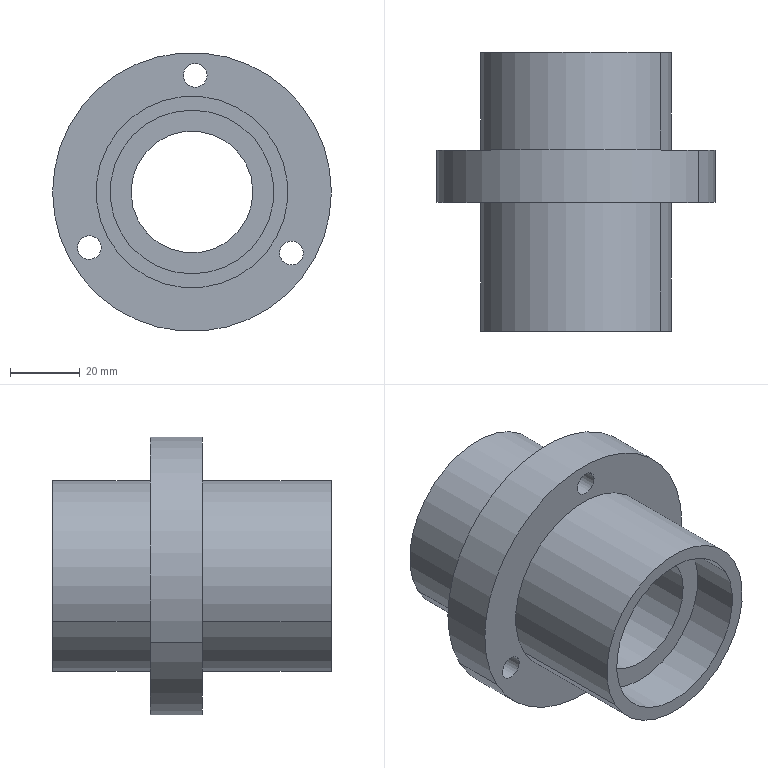Component | SolidWorks | BearingHousing1-1 | 1 solid | 24 faces | box 80 x 80 x 80 mm | volume 129585 mm3 | cylinder 18 | plane 6 | commonest cylinder face diameters 6.8 x6 47 x4 55 x4 35 x2 80 x2
STEP:
#1=CARTESIAN_POINT('',(-9.498,17.558,-6.667));
#2=VERTEX_POINT('',#1);
#3=CARTESIAN_POINT('',(-9.733,17.558,-6.794));
#4=VERTEX_POINT('',#3);
#5=CARTESIAN_POINT('',(-9.616,17.558,-6.73));
#6=DIRECTION('',(0.,-1.,0.));
#7=DIRECTION('',(-0.8793,0.,-0.4762));
#8=AXIS2_PLACEMENT_3D('',#5,#6,#7);
#9=CIRCLE('',#8,0.1339);
#10=EDGE_CURVE('',#2,#4,#9,.T.);
#11=ORIENTED_EDGE('',*,*,#10,.T.);
#12=CARTESIAN_POINT('',(-9.733,18.149,-6.794));
#13=VERTEX_POINT('',#12);
#14=CARTESIAN_POINT('',(-9.733,18.149,-6.794));
#15=DIRECTION('',(0.,1.,0.));
#16=VECTOR('',#15,39.37);
#17=LINE('',#14,#16);
#18=EDGE_CURVE('',#4,#13,#17,.T.);
#19=ORIENTED_EDGE('',*,*,#18,.T.);
#20=CARTESIAN_POINT('',(-9.498,18.149,-6.667));
#21=VERTEX_POINT('',#20);
#22=CARTESIAN_POINT('',(-9.616,18.149,-6.73));
#23=DIRECTION('',(0.,1.,0.));
#24=DIRECTION('',(0.8793,0.,0.4762));
#25=AXIS2_PLACEMENT_3D('',#22,#23,#24);
#26=CIRCLE('',#25,0.1339);
#27=EDGE_CURVE('',#13,#21,#26,.T.);
#28=ORIENTED_EDGE('',*,*,#27,.T.);
#29=CARTESIAN_POINT('',(-9.498,18.149,-6.667));
#30=DIRECTION('',(0.,1.,0.));
#31=VECTOR('',#30,39.37);
#32=LINE('',#29,#31);
#33=EDGE_CURVE('',#2,#21,#32,.T.);
#34=ORIENTED_EDGE('',*,*,#33,.F.);
#35=EDGE_LOOP('',(#11,#19,#28,#34));
#36=FACE_OUTER_BOUND('',#35,.T.);
#37=CARTESIAN_POINT('',(-9.616,18.149,-6.73));
#38=DIRECTION('',(0.,1.,0.));
#39=DIRECTION('',(0.8793,0.,0.4762));
#40=AXIS2_PLACEMENT_3D('',#37,#38,#39);
#41=CYLINDRICAL_SURFACE('',#40,0.1339);
#42=ADVANCED_FACE('',(#36),#41,.F.);
#43=CARTESIAN_POINT('',(-8.302,17.558,-4.72));
#44=VERTEX_POINT('',#43);
#45=CARTESIAN_POINT('',(-8.538,17.558,-4.848));
#46=VERTEX_POINT('',#45);
#47=CARTESIAN_POINT('',(-8.42,17.558,-4.784));
#48=DIRECTION('',(0.,-1.,0.));
#49=DIRECTION('',(-0.8793,0.,-0.4762));
#50=AXIS2_PLACEMENT_3D('',#47,#48,#49);
#51=CIRCLE('',#50,0.1339);
#52=EDGE_CURVE('',#44,#46,#51,.T.);
#53=ORIENTED_EDGE('',*,*,#52,.T.);
#54=CARTESIAN_POINT('',(-8.538,18.149,-4.848));
#55=VERTEX_POINT('',#54);
#56=CARTESIAN_POINT('',(-8.538,18.149,-4.848));
#57=DIRECTION('',(0.,1.,0.));
#58=VECTOR('',#57,39.37);
#59=LINE('',#56,#58);
#60=EDGE_CURVE('',#46,#55,#59,.T.);
#61=ORIENTED_EDGE('',*,*,#60,.T.);
#62=CARTESIAN_POINT('',(-8.302,18.149,-4.72));
#63=VERTEX_POINT('',#62);
#64=CARTESIAN_POINT('',(-8.42,18.149,-4.784));
#65=DIRECTION('',(0.,1.,0.));
#66=DIRECTION('',(0.8793,0.,0.4762));
#67=AXIS2_PLACEMENT_3D('',#64,#65,#66);
#68=CIRCLE('',#67,0.1339);
#69=EDGE_CURVE('',#55,#63,#68,.T.);
#70=ORIENTED_EDGE('',*,*,#69,.T.);
#71=CARTESIAN_POINT('',(-8.302,18.149,-4.72));
#72=DIRECTION('',(0.,1.,0.));
#73=VECTOR('',#72,39.37);
#74=LINE('',#71,#73);
#75=EDGE_CURVE('',#44,#63,#74,.T.);
#76=ORIENTED_EDGE('',*,*,#75,.F.);
#77=EDGE_LOOP('',(#53,#61,#70,#76));
#78=FACE_OUTER_BOUND('',#77,.T.);
#79=CARTESIAN_POINT('',(-8.42,18.149,-4.784));
#80=DIRECTION('',(0.,1.,0.));
#81=DIRECTION('',(0.8793,0.,0.4762));
#82=AXIS2_PLACEMENT_3D('',#79,#80,#81);
#83=CYLINDRICAL_SURFACE('',#82,0.1339);
#84=ADVANCED_FACE('',(#78),#83,.F.);
#85=CARTESIAN_POINT('',(-7.215,17.558,-6.729));
#86=VERTEX_POINT('',#85);
#87=CARTESIAN_POINT('',(-7.45,17.558,-6.856));
#88=VERTEX_POINT('',#87);
#89=CARTESIAN_POINT('',(-7.332,17.558,-6.793));
#90=DIRECTION('',(0.,-1.,0.));
#91=DIRECTION('',(-0.8793,0.,-0.4762));
#92=AXIS2_PLACEMENT_3D('',#89,#90,#91);
#93=CIRCLE('',#92,0.1339);
#94=EDGE_CURVE('',#86,#88,#93,.T.);
#95=ORIENTED_EDGE('',*,*,#94,.T.);
#96=CARTESIAN_POINT('',(-7.45,18.149,-6.856));
#97=VERTEX_POINT('',#96);
#98=CARTESIAN_POINT('',(-7.45,18.149,-6.856));
#99=DIRECTION('',(0.,1.,0.));
#100=VECTOR('',#99,39.37);
#101=LINE('',#98,#100);
#102=EDGE_CURVE('',#88,#97,#101,.T.);
#103=ORIENTED_EDGE('',*,*,#102,.T.);
#104=CARTESIAN_POINT('',(-7.215,18.149,-6.729));
#105=VERTEX_POINT('',#104);
#106=CARTESIAN_POINT('',(-7.332,18.149,-6.793));
#107=DIRECTION('',(0.,1.,0.));
#108=DIRECTION('',(0.8793,0.,0.4762));
#109=AXIS2_PLACEMENT_3D('',#106,#107,#108);
#110=CIRCLE('',#109,0.1339);
#111=EDGE_CURVE('',#97,#105,#110,.T.);
#112=ORIENTED_EDGE('',*,*,#111,.T.);
#113=CARTESIAN_POINT('',(-7.215,18.149,-6.729));
#114=DIRECTION('',(0.,1.,0.));
#115=VECTOR('',#114,39.37);
#116=LINE('',#113,#115);
#117=EDGE_CURVE('',#86,#105,#116,.T.);
#118=ORIENTED_EDGE('',*,*,#117,.F.);
#119=EDGE_LOOP('',(#95,#103,#112,#118));
#120=FACE_OUTER_BOUND('',#119,.T.);
#121=CARTESIAN_POINT('',(-7.332,18.149,-6.793));
#122=DIRECTION('',(0.,1.,0.));
#123=DIRECTION('',(0.8793,0.,0.4762));
#124=AXIS2_PLACEMENT_3D('',#121,#122,#123);
#125=CYLINDRICAL_SURFACE('',#124,0.1339);
#126=ADVANCED_FACE('',(#120),#125,.F.);
#127=CARTESIAN_POINT('',(-7.85,18.7,-5.774));
#128=VERTEX_POINT('',#127);
#129=CARTESIAN_POINT('',(-9.062,18.7,-6.43));
#130=VERTEX_POINT('',#129);
#131=CARTESIAN_POINT('',(-8.456,18.7,-6.102));
#132=DIRECTION('',(0.,-1.,0.));
#133=DIRECTION('',(-0.8793,0.,-0.4762));
#134=AXIS2_PLACEMENT_3D('',#131,#132,#133);
#135=CIRCLE('',#134,0.689);
#136=EDGE_CURVE('',#128,#130,#135,.T.);
#137=ORIENTED_EDGE('',*,*,#136,.F.);
#138=CARTESIAN_POINT('',(-7.85,16.653,-5.774));
#139=VERTEX_POINT('',#138);
#140=CARTESIAN_POINT('',(-7.85,17.335,-5.774));
#141=DIRECTION('',(0.,-1.,0.));
#142=VECTOR('',#141,39.37);
#143=LINE('',#140,#142);
#144=EDGE_CURVE('',#128,#139,#143,.T.);
#145=ORIENTED_EDGE('',*,*,#144,.T.);
#146=CARTESIAN_POINT('',(-9.062,16.653,-6.43));
#147=VERTEX_POINT('',#146);
#148=CARTESIAN_POINT('',(-8.456,16.653,-6.102));
#149=DIRECTION('',(0.,-1.,0.));
#150=DIRECTION('',(-0.8793,0.,-0.4762));
#151=AXIS2_PLACEMENT_3D('',#148,#149,#150);
#152=CIRCLE('',#151,0.689);
#153=EDGE_CURVE('',#139,#147,#152,.T.);
#154=ORIENTED_EDGE('',*,*,#153,.T.);
#155=CARTESIAN_POINT('',(-9.062,17.335,-6.43));
#156=DIRECTION('',(0.,-1.,0.));
#157=VECTOR('',#156,39.37);
#158=LINE('',#155,#157);
#159=EDGE_CURVE('',#130,#147,#158,.T.);
#160=ORIENTED_EDGE('',*,*,#159,.F.);
#161=EDGE_LOOP('',(#137,#145,#154,#160));
#162=FACE_OUTER_BOUND('',#161,.T.);
#163=CARTESIAN_POINT('',(-8.456,17.335,-6.102));
#164=DIRECTION('',(0.,-1.,0.));
#165=DIRECTION('',(-0.8793,0.,-0.4762));
#166=AXIS2_PLACEMENT_3D('',#163,#164,#165);
#167=CYLINDRICAL_SURFACE('',#166,0.689);
#168=ADVANCED_FACE('',(#162),#167,.F.);
#169=CARTESIAN_POINT('',(-7.643,19.251,-5.662));
#170=VERTEX_POINT('',#169);
#171=CARTESIAN_POINT('',(-9.27,19.251,-6.543));
#172=VERTEX_POINT('',#171);
#173=CARTESIAN_POINT('',(-8.456,19.251,-6.102));
#174=DIRECTION('',(0.,-1.,0.));
#175=DIRECTION('',(-0.8793,0.,-0.4762));
#176=AXIS2_PLACEMENT_3D('',#173,#174,#175);
#177=CIRCLE('',#176,0.9252);
#178=EDGE_CURVE('',#170,#172,#177,.T.);
#179=ORIENTED_EDGE('',*,*,#178,.F.);
#180=CARTESIAN_POINT('',(-7.643,18.7,-5.662));
#181=VERTEX_POINT('',#180);
#182=CARTESIAN_POINT('',(-7.643,17.335,-5.662));
#183=DIRECTION('',(0.,-1.,0.));
#184=VECTOR('',#183,39.37);
#185=LINE('',#182,#184);
#186=EDGE_CURVE('',#170,#181,#185,.T.);
#187=ORIENTED_EDGE('',*,*,#186,.T.);
#188=CARTESIAN_POINT('',(-9.27,18.7,-6.543));
#189=VERTEX_POINT('',#188);
#190=CARTESIAN_POINT('',(-8.456,18.7,-6.102));
#191=DIRECTION('',(0.,-1.,0.));
#192=DIRECTION('',(-0.8793,0.,-0.4762));
#193=AXIS2_PLACEMENT_3D('',#190,#191,#192);
#194=CIRCLE('',#193,0.9252);
#195=EDGE_CURVE('',#181,#189,#194,.T.);
#196=ORIENTED_EDGE('',*,*,#195,.T.);
#197=CARTESIAN_POINT('',(-9.27,17.335,-6.543));
#198=DIRECTION('',(0.,-1.,0.));
#199=VECTOR('',#198,39.37);
#200=LINE('',#197,#199);
#201=EDGE_CURVE('',#172,#189,#200,.T.);
#202=ORIENTED_EDGE('',*,*,#201,.F.);
#203=EDGE_LOOP('',(#179,#187,#196,#202));
#204=FACE_OUTER_BOUND('',#203,.T.);
#205=CARTESIAN_POINT('',(-8.456,17.335,-6.102));
#206=DIRECTION('',(0.,-1.,0.));
#207=DIRECTION('',(-0.8793,0.,-0.4762));
#208=AXIS2_PLACEMENT_3D('',#205,#206,#207);
#209=CYLINDRICAL_SURFACE('',#208,0.9252);
#210=ADVANCED_FACE('',(#204),#209,.F.);
#211=CARTESIAN_POINT('',(-9.408,19.251,-6.618));
#212=VERTEX_POINT('',#211);
#213=CARTESIAN_POINT('',(-7.504,19.251,-5.587));
#214=VERTEX_POINT('',#213);
#215=CARTESIAN_POINT('',(-8.456,19.251,-6.102));
#216=DIRECTION('',(0.,-1.,0.));
#217=DIRECTION('',(-0.8793,0.,-0.4762));
#218=AXIS2_PLACEMENT_3D('',#215,#216,#217);
#219=CIRCLE('',#218,1.083);
#220=EDGE_CURVE('',#212,#214,#219,.T.);
#221=ORIENTED_EDGE('',*,*,#220,.T.);
#222=CARTESIAN_POINT('',(-7.504,18.149,-5.587));
#223=VERTEX_POINT('',#222);
#224=CARTESIAN_POINT('',(-7.504,17.335,-5.587));
#225=DIRECTION('',(0.,-1.,0.));
#226=VECTOR('',#225,39.37);
#227=LINE('',#224,#226);
#228=EDGE_CURVE('',#214,#223,#227,.T.);
#229=ORIENTED_EDGE('',*,*,#228,.T.);
#230=CARTESIAN_POINT('',(-9.408,18.149,-6.618));
#231=VERTEX_POINT('',#230);
#232=CARTESIAN_POINT('',(-8.456,18.149,-6.102));
#233=DIRECTION('',(0.,-1.,0.));
#234=DIRECTION('',(-0.8793,0.,-0.4762));
#235=AXIS2_PLACEMENT_3D('',#232,#233,#234);
#236=CIRCLE('',#235,1.083);
#237=EDGE_CURVE('',#231,#223,#236,.T.);
#238=ORIENTED_EDGE('',*,*,#237,.F.);
#239=CARTESIAN_POINT('',(-9.408,17.335,-6.618));
#240=DIRECTION('',(0.,-1.,0.));
#241=VECTOR('',#240,39.37);
#242=LINE('',#239,#241);
#243=EDGE_CURVE('',#212,#231,#242,.T.);
#244=ORIENTED_EDGE('',*,*,#243,.F.);
#245=EDGE_LOOP('',(#221,#229,#238,#244));
#246=FACE_OUTER_BOUND('',#245,.T.);
#247=CARTESIAN_POINT('',(-8.456,17.335,-6.102));
#248=DIRECTION('',(0.,-1.,0.));
#249=DIRECTION('',(-0.8793,0.,-0.4762));
#250=AXIS2_PLACEMENT_3D('',#247,#248,#249);
#251=CYLINDRICAL_SURFACE('',#250,1.083);
#252=ADVANCED_FACE('',(#246),#251,.T.);
#253=CARTESIAN_POINT('',(-9.841,18.149,-6.852));
#254=VERTEX_POINT('',#253);
#255=CARTESIAN_POINT('',(-7.071,18.149,-5.352));
#256=VERTEX_POINT('',#255);
#257=CARTESIAN_POINT('',(-8.456,18.149,-6.102));
#258=DIRECTION('',(0.,-1.,0.));
#259=DIRECTION('',(-0.8793,0.,-0.4762));
#260=AXIS2_PLACEMENT_3D('',#257,#258,#259);
#261=CIRCLE('',#260,1.575);
#262=EDGE_CURVE('',#254,#256,#261,.T.);
#263=ORIENTED_EDGE('',*,*,#262,.T.);
#264=CARTESIAN_POINT('',(-7.071,17.558,-5.352));
#265=VERTEX_POINT('',#264);
#266=CARTESIAN_POINT('',(-7.071,17.335,-5.352));
#267=DIRECTION('',(0.,-1.,0.));
#268=VECTOR('',#267,39.37);
#269=LINE('',#266,#268);
#270=EDGE_CURVE('',#256,#265,#269,.T.);
#271=ORIENTED_EDGE('',*,*,#270,.T.);
#272=CARTESIAN_POINT('',(-9.841,17.558,-6.852));
#273=VERTEX_POINT('',#272);
#274=CARTESIAN_POINT('',(-8.456,17.558,-6.102));
#275=DIRECTION('',(0.,-1.,0.));
#276=DIRECTION('',(-0.8793,0.,-0.4762));
#277=AXIS2_PLACEMENT_3D('',#274,#275,#276);
#278=CIRCLE('',#277,1.575);
#279=EDGE_CURVE('',#273,#265,#278,.T.);
#280=ORIENTED_EDGE('',*,*,#279,.F.);
#281=CARTESIAN_POINT('',(-9.841,17.335,-6.852));
#282=DIRECTION('',(0.,-1.,0.));
#283=VECTOR('',#282,39.37);
#284=LINE('',#281,#283);
#285=EDGE_CURVE('',#254,#273,#284,.T.);
#286=ORIENTED_EDGE('',*,*,#285,.F.);
#287=EDGE_LOOP('',(#263,#271,#280,#286));
#288=FACE_OUTER_BOUND('',#287,.T.);
#289=CARTESIAN_POINT('',(-8.456,17.335,-6.102));
#290=DIRECTION('',(0.,-1.,0.));
#291=DIRECTION('',(-0.8793,0.,-0.4762));
#292=AXIS2_PLACEMENT_3D('',#289,#290,#291);
#293=CYLINDRICAL_SURFACE('',#292,1.575);
#294=ADVANCED_FACE('',(#288),#293,.T.);
#295=CARTESIAN_POINT('',(-9.408,17.558,-6.618));
#296=VERTEX_POINT('',#295);
#297=CARTESIAN_POINT('',(-7.504,17.558,-5.587));
#298=VERTEX_POINT('',#297);
#299=CARTESIAN_POINT('',(-8.456,17.558,-6.102));
#300=DIRECTION('',(0.,-1.,0.));
#301=DIRECTION('',(-0.8793,0.,-0.4762));
#302=AXIS2_PLACEMENT_3D('',#299,#300,#301);
#303=CIRCLE('',#302,1.083);
#304=EDGE_CURVE('',#296,#298,#303,.T.);
#305=ORIENTED_EDGE('',*,*,#304,.T.);
#306=CARTESIAN_POINT('',(-7.504,16.102,-5.587));
#307=VERTEX_POINT('',#306);
#308=CARTESIAN_POINT('',(-7.504,17.335,-5.587));
#309=DIRECTION('',(0.,-1.,0.));
#310=VECTOR('',#309,39.37);
#311=LINE('',#308,#310);
#312=EDGE_CURVE('',#298,#307,#311,.T.);
#313=ORIENTED_EDGE('',*,*,#312,.T.);
#314=CARTESIAN_POINT('',(-9.408,16.102,-6.618));
#315=VERTEX_POINT('',#314);
#316=CARTESIAN_POINT('',(-8.456,16.102,-6.102));
#317=DIRECTION('',(0.,-1.,0.));
#318=DIRECTION('',(-0.8793,0.,-0.4762));
#319=AXIS2_PLACEMENT_3D('',#316,#317,#318);
#320=CIRCLE('',#319,1.083);
#321=EDGE_CURVE('',#315,#307,#320,.T.);
#322=ORIENTED_EDGE('',*,*,#321,.F.);
#323=CARTESIAN_POINT('',(-9.408,17.335,-6.618));
#324=DIRECTION('',(0.,-1.,0.));
#325=VECTOR('',#324,39.37);
#326=LINE('',#323,#325);
#327=EDGE_CURVE('',#296,#315,#326,.T.);
#328=ORIENTED_EDGE('',*,*,#327,.F.);
#329=EDGE_LOOP('',(#305,#313,#322,#328));
#330=FACE_OUTER_BOUND('',#329,.T.);
#331=CARTESIAN_POINT('',(-8.456,17.335,-6.102));
#332=DIRECTION('',(0.,-1.,0.));
#333=DIRECTION('',(-0.8793,0.,-0.4762));
#334=AXIS2_PLACEMENT_3D('',#331,#332,#333);
#335=CYLINDRICAL_SURFACE('',#334,1.083);
#336=ADVANCED_FACE('',(#330),#335,.T.);
#337=CARTESIAN_POINT('',(-7.643,16.653,-5.662));
#338=VERTEX_POINT('',#337);
#339=CARTESIAN_POINT('',(-9.27,16.653,-6.543));
#340=VERTEX_POINT('',#339);
#341=CARTESIAN_POINT('',(-8.456,16.653,-6.102));
#342=DIRECTION('',(0.,-1.,0.));
#343=DIRECTION('',(-0.8793,0.,-0.4762));
#344=AXIS2_PLACEMENT_3D('',#341,#342,#343);
#345=CIRCLE('',#344,0.9252);
#346=EDGE_CURVE('',#338,#340,#345,.T.);
#347=ORIENTED_EDGE('',*,*,#346,.F.);
#348=CARTESIAN_POINT('',(-7.643,16.102,-5.662));
#349=VERTEX_POINT('',#348);
#350=CARTESIAN_POINT('',(-7.643,17.335,-5.662));
#351=DIRECTION('',(0.,-1.,0.));
#352=VECTOR('',#351,39.37);
#353=LINE('',#350,#352);
#354=EDGE_CURVE('',#338,#349,#353,.T.);
#355=ORIENTED_EDGE('',*,*,#354,.T.);
#356=CARTESIAN_POINT('',(-9.27,16.102,-6.543));
#357=VERTEX_POINT('',#356);
#358=CARTESIAN_POINT('',(-8.456,16.102,-6.102));
#359=DIRECTION('',(0.,-1.,0.));
#360=DIRECTION('',(-0.8793,0.,-0.4762));
#361=AXIS2_PLACEMENT_3D('',#358,#359,#360);
#362=CIRCLE('',#361,0.9252);
#363=EDGE_CURVE('',#349,#357,#362,.T.);
#364=ORIENTED_EDGE('',*,*,#363,.T.);
#365=CARTESIAN_POINT('',(-9.27,17.335,-6.543));
#366=DIRECTION('',(0.,-1.,0.));
#367=VECTOR('',#366,39.37);
#368=LINE('',#365,#367);
#369=EDGE_CURVE('',#340,#357,#368,.T.);
#370=ORIENTED_EDGE('',*,*,#369,.F.);
#371=EDGE_LOOP('',(#347,#355,#364,#370));
#372=FACE_OUTER_BOUND('',#371,.T.);
#373=CARTESIAN_POINT('',(-8.456,17.335,-6.102));
#374=DIRECTION('',(0.,-1.,0.));
#375=DIRECTION('',(-0.8793,0.,-0.4762));
#376=AXIS2_PLACEMENT_3D('',#373,#374,#375);
#377=CYLINDRICAL_SURFACE('',#376,0.9252);
#378=ADVANCED_FACE('',(#372),#377,.F.);
#379=ORIENTED_EDGE('',*,*,#354,.F.);
#380=CARTESIAN_POINT('',(-8.456,16.653,-6.102));
#381=DIRECTION('',(0.,-1.,0.));
#382=DIRECTION('',(-0.8793,0.,-0.4762));
#383=AXIS2_PLACEMENT_3D('',#380,#381,#382);
#384=CIRCLE('',#383,0.9252);
#385=EDGE_CURVE('',#340,#338,#384,.T.);
#386=ORIENTED_EDGE('',*,*,#385,.F.);
#387=ORIENTED_EDGE('',*,*,#369,.T.);
#388=CARTESIAN_POINT('',(-8.456,16.102,-6.102));
#389=DIRECTION('',(0.,-1.,0.));
#390=DIRECTION('',(-0.8793,0.,-0.4762));
#391=AXIS2_PLACEMENT_3D('',#388,#389,#390);
#392=CIRCLE('',#391,0.9252);
#393=EDGE_CURVE('',#357,#349,#392,.T.);
#394=ORIENTED_EDGE('',*,*,#393,.T.);
#395=EDGE_LOOP('',(#379,#386,#387,#394));
#396=FACE_OUTER_BOUND('',#395,.T.);
#397=CARTESIAN_POINT('',(-8.456,17.335,-6.102));
#398=DIRECTION('',(0.,-1.,0.));
#399=DIRECTION('',(-0.8793,0.,-0.4762));
#400=AXIS2_PLACEMENT_3D('',#397,#398,#399);
#401=CYLINDRICAL_SURFACE('',#400,0.9252);
#402=ADVANCED_FACE('',(#396),#401,.F.);
#403=ORIENTED_EDGE('',*,*,#321,.T.);
#404=CARTESIAN_POINT('',(-8.456,16.102,-6.102));
#405=DIRECTION('',(0.,-1.,0.));
#406=DIRECTION('',(-0.8793,0.,-0.4762));
#407=AXIS2_PLACEMENT_3D('',#404,#405,#406);
#408=CIRCLE('',#407,1.083);
#409=EDGE_CURVE('',#307,#315,#408,.T.);
#410=ORIENTED_EDGE('',*,*,#409,.T.);
#411=EDGE_LOOP('',(#403,#410));
#412=FACE_OUTER_BOUND('',#411,.T.);
#413=ORIENTED_EDGE('',*,*,#393,.F.);
#414=ORIENTED_EDGE('',*,*,#363,.F.);
#415=EDGE_LOOP('',(#413,#414));
#416=FACE_BOUND('',#415,.T.);
#417=CARTESIAN_POINT('',(-9.408,16.102,-6.618));
#418=DIRECTION('',(0.,-1.,0.));
#419=DIRECTION('',(-0.8793,-0.,-0.4762));
#420=AXIS2_PLACEMENT_3D('',#417,#418,#419);
#421=PLANE('',#420);
#422=ADVANCED_FACE('',(#412,#416),#421,.T.);
#423=ORIENTED_EDGE('',*,*,#312,.F.);
#424=CARTESIAN_POINT('',(-8.456,17.558,-6.102));
#425=DIRECTION('',(0.,-1.,0.));
#426=DIRECTION('',(-0.8793,0.,-0.4762));
#427=AXIS2_PLACEMENT_3D('',#424,#425,#426);
#428=CIRCLE('',#427,1.083);
#429=EDGE_CURVE('',#298,#296,#428,.T.);
#430=ORIENTED_EDGE('',*,*,#429,.T.);
#431=ORIENTED_EDGE('',*,*,#327,.T.);
#432=ORIENTED_EDGE('',*,*,#409,.F.);
#433=EDGE_LOOP('',(#423,#430,#431,#432));
#434=FACE_OUTER_BOUND('',#433,.T.);
#435=CARTESIAN_POINT('',(-8.456,17.335,-6.102));
#436=DIRECTION('',(0.,-1.,0.));
#437=DIRECTION('',(-0.8793,0.,-0.4762));
#438=AXIS2_PLACEMENT_3D('',#435,#436,#437);
#439=CYLINDRICAL_SURFACE('',#438,1.083);
#440=ADVANCED_FACE('',(#434),#439,.T.);
#441=ORIENTED_EDGE('',*,*,#10,.F.);
#442=CARTESIAN_POINT('',(-9.616,17.558,-6.73));
#443=DIRECTION('',(0.,-1.,0.));
#444=DIRECTION('',(-0.8793,0.,-0.4762));
#445=AXIS2_PLACEMENT_3D('',#442,#443,#444);
#446=CIRCLE('',#445,0.1339);
#447=EDGE_CURVE('',#4,#2,#446,.T.);
#448=ORIENTED_EDGE('',*,*,#447,.F.);
#449=EDGE_LOOP('',(#441,#448));
#450=FACE_BOUND('',#449,.T.);
#451=ORIENTED_EDGE('',*,*,#52,.F.);
#452=CARTESIAN_POINT('',(-8.42,17.558,-4.784));
#453=DIRECTION('',(0.,-1.,0.));
#454=DIRECTION('',(-0.8793,0.,-0.4762));
#455=AXIS2_PLACEMENT_3D('',#452,#453,#454);
#456=CIRCLE('',#455,0.1339);
#457=EDGE_CURVE('',#46,#44,#456,.T.);
#458=ORIENTED_EDGE('',*,*,#457,.F.);
#459=EDGE_LOOP('',(#451,#458));
#460=FACE_BOUND('',#459,.T.);
#461=ORIENTED_EDGE('',*,*,#94,.F.);
#462=CARTESIAN_POINT('',(-7.332,17.558,-6.793));
#463=DIRECTION('',(0.,-1.,0.));
#464=DIRECTION('',(-0.8793,0.,-0.4762));
#465=AXIS2_PLACEMENT_3D('',#462,#463,#464);
#466=CIRCLE('',#465,0.1339);
#467=EDGE_CURVE('',#88,#86,#466,.T.);
#468=ORIENTED_EDGE('',*,*,#467,.F.);
#469=EDGE_LOOP('',(#461,#468));
#470=FACE_BOUND('',#469,.T.);
#471=ORIENTED_EDGE('',*,*,#279,.T.);
#472=CARTESIAN_POINT('',(-8.456,17.558,-6.102));
#473=DIRECTION('',(0.,-1.,0.));
#474=DIRECTION('',(-0.8793,0.,-0.4762));
#475=AXIS2_PLACEMENT_3D('',#472,#473,#474);
#476=CIRCLE('',#475,1.575);
#477=EDGE_CURVE('',#265,#273,#476,.T.);
#478=ORIENTED_EDGE('',*,*,#477,.T.);
#479=EDGE_LOOP('',(#471,#478));
#480=FACE_OUTER_BOUND('',#479,.T.);
#481=ORIENTED_EDGE('',*,*,#304,.F.);
#482=ORIENTED_EDGE('',*,*,#429,.F.);
#483=EDGE_LOOP('',(#481,#482));
#484=FACE_BOUND('',#483,.T.);
#485=CARTESIAN_POINT('',(-9.841,17.558,-6.852));
#486=DIRECTION('',(0.,-1.,0.));
#487=DIRECTION('',(-0.8793,-0.,-0.4762));
#488=AXIS2_PLACEMENT_3D('',#485,#486,#487);
#489=PLANE('',#488);
#490=ADVANCED_FACE('',(#450,#460,#470,#480,#484),#489,.T.);
#491=ORIENTED_EDGE('',*,*,#270,.F.);
#492=CARTESIAN_POINT('',(-8.456,18.149,-6.102));
#493=DIRECTION('',(0.,-1.,0.));
#494=DIRECTION('',(-0.8793,0.,-0.4762));
#495=AXIS2_PLACEMENT_3D('',#492,#493,#494);
#496=CIRCLE('',#495,1.575);
#497=EDGE_CURVE('',#256,#254,#496,.T.);
#498=ORIENTED_EDGE('',*,*,#497,.T.);
#499=ORIENTED_EDGE('',*,*,#285,.T.);
#500=ORIENTED_EDGE('',*,*,#477,.F.);
#501=EDGE_LOOP('',(#491,#498,#499,#500));
#502=FACE_OUTER_BOUND('',#501,.T.);
#503=CARTESIAN_POINT('',(-8.456,17.335,-6.102));
#504=DIRECTION('',(0.,-1.,0.));
#505=DIRECTION('',(-0.8793,0.,-0.4762));
#506=AXIS2_PLACEMENT_3D('',#503,#504,#505);
#507=CYLINDRICAL_SURFACE('',#506,1.575);
#508=ADVANCED_FACE('',(#502),#507,.T.);
#509=CARTESIAN_POINT('',(-9.616,18.149,-6.73));
#510=DIRECTION('',(0.,1.,0.));
#511=DIRECTION('',(0.8793,0.,0.4762));
#512=AXIS2_PLACEMENT_3D('',#509,#510,#511);
#513=CIRCLE('',#512,0.1339);
#514=EDGE_CURVE('',#21,#13,#513,.T.);
#515=ORIENTED_EDGE('',*,*,#514,.F.);
#516=ORIENTED_EDGE('',*,*,#27,.F.);
#517=EDGE_LOOP('',(#515,#516));
#518=FACE_BOUND('',#517,.T.);
#519=CARTESIAN_POINT('',(-8.42,18.149,-4.784));
#520=DIRECTION('',(0.,1.,0.));
#521=DIRECTION('',(0.8793,0.,0.4762));
#522=AXIS2_PLACEMENT_3D('',#519,#520,#521);
#523=CIRCLE('',#522,0.1339);
#524=EDGE_CURVE('',#63,#55,#523,.T.);
#525=ORIENTED_EDGE('',*,*,#524,.F.);
#526=ORIENTED_EDGE('',*,*,#69,.F.);
#527=EDGE_LOOP('',(#525,#526));
#528=FACE_BOUND('',#527,.T.);
#529=CARTESIAN_POINT('',(-7.332,18.149,-6.793));
#530=DIRECTION('',(0.,1.,0.));
#531=DIRECTION('',(0.8793,0.,0.4762));
#532=AXIS2_PLACEMENT_3D('',#529,#530,#531);
#533=CIRCLE('',#532,0.1339);
#534=EDGE_CURVE('',#105,#97,#533,.T.);
#535=ORIENTED_EDGE('',*,*,#534,.F.);
#536=ORIENTED_EDGE('',*,*,#111,.F.);
#537=EDGE_LOOP('',(#535,#536));
#538=FACE_BOUND('',#537,.T.);
#539=ORIENTED_EDGE('',*,*,#237,.T.);
#540=CARTESIAN_POINT('',(-8.456,18.149,-6.102));
#541=DIRECTION('',(0.,-1.,0.));
#542=DIRECTION('',(-0.8793,0.,-0.4762));
#543=AXIS2_PLACEMENT_3D('',#540,#541,#542);
#544=CIRCLE('',#543,1.083);
#545=EDGE_CURVE('',#223,#231,#544,.T.);
#546=ORIENTED_EDGE('',*,*,#545,.T.);
#547=EDGE_LOOP('',(#539,#546));
#548=FACE_BOUND('',#547,.T.);
#549=ORIENTED_EDGE('',*,*,#262,.F.);
#550=ORIENTED_EDGE('',*,*,#497,.F.);
#551=EDGE_LOOP('',(#549,#550));
#552=FACE_OUTER_BOUND('',#551,.T.);
#553=CARTESIAN_POINT('',(-9.408,18.149,-6.618));
#554=DIRECTION('',(-0.,1.,-0.));
#555=DIRECTION('',(0.8793,0.,0.4762));
#556=AXIS2_PLACEMENT_3D('',#553,#554,#555);
#557=PLANE('',#556);
#558=ADVANCED_FACE('',(#518,#528,#538,#548,#552),#557,.T.);
#559=ORIENTED_EDGE('',*,*,#228,.F.);
#560=CARTESIAN_POINT('',(-8.456,19.251,-6.102));
#561=DIRECTION('',(0.,-1.,0.));
#562=DIRECTION('',(-0.8793,0.,-0.4762));
#563=AXIS2_PLACEMENT_3D('',#560,#561,#562);
#564=CIRCLE('',#563,1.083);
#565=EDGE_CURVE('',#214,#212,#564,.T.);
#566=ORIENTED_EDGE('',*,*,#565,.T.);
#567=ORIENTED_EDGE('',*,*,#243,.T.);
#568=ORIENTED_EDGE('',*,*,#545,.F.);
#569=EDGE_LOOP('',(#559,#566,#567,#568));
#570=FACE_OUTER_BOUND('',#569,.T.);
#571=CARTESIAN_POINT('',(-8.456,17.335,-6.102));
#572=DIRECTION('',(0.,-1.,0.));
#573=DIRECTION('',(-0.8793,0.,-0.4762));
#574=AXIS2_PLACEMENT_3D('',#571,#572,#573);
#575=CYLINDRICAL_SURFACE('',#574,1.083);
#576=ADVANCED_FACE('',(#570),#575,.T.);
#577=CARTESIAN_POINT('',(-8.456,19.251,-6.102));
#578=DIRECTION('',(0.,-1.,0.));
#579=DIRECTION('',(-0.8793,0.,-0.4762));
#580=AXIS2_PLACEMENT_3D('',#577,#578,#579);
#581=CIRCLE('',#580,0.9252);
#582=EDGE_CURVE('',#172,#170,#581,.T.);
#583=ORIENTED_EDGE('',*,*,#582,.T.);
#584=ORIENTED_EDGE('',*,*,#178,.T.);
#585=EDGE_LOOP('',(#583,#584));
#586=FACE_BOUND('',#585,.T.);
#587=ORIENTED_EDGE('',*,*,#220,.F.);
#588=ORIENTED_EDGE('',*,*,#565,.F.);
#589=EDGE_LOOP('',(#587,#588));
#590=FACE_OUTER_BOUND('',#589,.T.);
#591=CARTESIAN_POINT('',(-9.27,19.251,-6.543));
#592=DIRECTION('',(-0.,1.,-0.));
#593=DIRECTION('',(0.8793,0.,0.4762));
#594=AXIS2_PLACEMENT_3D('',#591,#592,#593);
#595=PLANE('',#594);
#596=ADVANCED_FACE('',(#586,#590),#595,.T.);
#597=ORIENTED_EDGE('',*,*,#186,.F.);
#598=ORIENTED_EDGE('',*,*,#582,.F.);
#599=ORIENTED_EDGE('',*,*,#201,.T.);
#600=CARTESIAN_POINT('',(-8.456,18.7,-6.102));
#601=DIRECTION('',(0.,-1.,0.));
#602=DIRECTION('',(-0.8793,0.,-0.4762));
#603=AXIS2_PLACEMENT_3D('',#600,#601,#602);
#604=CIRCLE('',#603,0.9252);
#605=EDGE_CURVE('',#189,#181,#604,.T.);
#606=ORIENTED_EDGE('',*,*,#605,.T.);
#607=EDGE_LOOP('',(#597,#598,#599,#606));
#608=FACE_OUTER_BOUND('',#607,.T.);
#609=CARTESIAN_POINT('',(-8.456,17.335,-6.102));
#610=DIRECTION('',(0.,-1.,0.));
#611=DIRECTION('',(-0.8793,0.,-0.4762));
#612=AXIS2_PLACEMENT_3D('',#609,#610,#611);
#613=CYLINDRICAL_SURFACE('',#612,0.9252);
#614=ADVANCED_FACE('',(#608),#613,.F.);
#615=CARTESIAN_POINT('',(-8.456,18.7,-6.102));
#616=DIRECTION('',(0.,-1.,0.));
#617=DIRECTION('',(-0.8793,0.,-0.4762));
#618=AXIS2_PLACEMENT_3D('',#615,#616,#617);
#619=CIRCLE('',#618,0.689);
#620=EDGE_CURVE('',#130,#128,#619,.T.);
#621=ORIENTED_EDGE('',*,*,#620,.T.);
#622=ORIENTED_EDGE('',*,*,#136,.T.);
#623=EDGE_LOOP('',(#621,#622));
#624=FACE_BOUND('',#623,.T.);
#625=ORIENTED_EDGE('',*,*,#605,.F.);
#626=ORIENTED_EDGE('',*,*,#195,.F.);
#627=EDGE_LOOP('',(#625,#626));
#628=FACE_OUTER_BOUND('',#627,.T.);
#629=CARTESIAN_POINT('',(-9.27,18.7,-6.543));
#630=DIRECTION('',(-0.,1.,-0.));
#631=DIRECTION('',(0.8793,0.,0.4762));
#632=AXIS2_PLACEMENT_3D('',#629,#630,#631);
#633=PLANE('',#632);
#634=ADVANCED_FACE('',(#624,#628),#633,.T.);
#635=ORIENTED_EDGE('',*,*,#144,.F.);
#636=ORIENTED_EDGE('',*,*,#620,.F.);
#637=ORIENTED_EDGE('',*,*,#159,.T.);
#638=CARTESIAN_POINT('',(-8.456,16.653,-6.102));
#639=DIRECTION('',(0.,-1.,0.));
#640=DIRECTION('',(-0.8793,0.,-0.4762));
#641=AXIS2_PLACEMENT_3D('',#638,#639,#640);
#642=CIRCLE('',#641,0.689);
#643=EDGE_CURVE('',#147,#139,#642,.T.);
#644=ORIENTED_EDGE('',*,*,#643,.T.);
#645=EDGE_LOOP('',(#635,#636,#637,#644));
#646=FACE_OUTER_BOUND('',#645,.T.);
#647=CARTESIAN_POINT('',(-8.456,17.335,-6.102));
#648=DIRECTION('',(0.,-1.,0.));
#649=DIRECTION('',(-0.8793,0.,-0.4762));
#650=AXIS2_PLACEMENT_3D('',#647,#648,#649);
#651=CYLINDRICAL_SURFACE('',#650,0.689);
#652=ADVANCED_FACE('',(#646),#651,.F.);
#653=ORIENTED_EDGE('',*,*,#385,.T.);
#654=ORIENTED_EDGE('',*,*,#346,.T.);
#655=EDGE_LOOP('',(#653,#654));
#656=FACE_OUTER_BOUND('',#655,.T.);
#657=ORIENTED_EDGE('',*,*,#643,.F.);
#658=ORIENTED_EDGE('',*,*,#153,.F.);
#659=EDGE_LOOP('',(#657,#658));
#660=FACE_BOUND('',#659,.T.);
#661=CARTESIAN_POINT('',(-9.27,16.653,-6.543));
#662=DIRECTION('',(0.,-1.,0.));
#663=DIRECTION('',(-0.8793,-0.,-0.4762));
#664=AXIS2_PLACEMENT_3D('',#661,#662,#663);
#665=PLANE('',#664);
#666=ADVANCED_FACE('',(#656,#660),#665,.T.);
#667=ORIENTED_EDGE('',*,*,#102,.F.);
#668=ORIENTED_EDGE('',*,*,#467,.T.);
#669=ORIENTED_EDGE('',*,*,#117,.T.);
#670=ORIENTED_EDGE('',*,*,#534,.T.);
#671=EDGE_LOOP('',(#667,#668,#669,#670));
#672=FACE_OUTER_BOUND('',#671,.T.);
#673=CARTESIAN_POINT('',(-7.332,18.149,-6.793));
#674=DIRECTION('',(0.,1.,0.));
#675=DIRECTION('',(0.8793,0.,0.4762));
#676=AXIS2_PLACEMENT_3D('',#673,#674,#675);
#677=CYLINDRICAL_SURFACE('',#676,0.1339);
#678=ADVANCED_FACE('',(#672),#677,.F.);
#679=ORIENTED_EDGE('',*,*,#60,.F.);
#680=ORIENTED_EDGE('',*,*,#457,.T.);
#681=ORIENTED_EDGE('',*,*,#75,.T.);
#682=ORIENTED_EDGE('',*,*,#524,.T.);
#683=EDGE_LOOP('',(#679,#680,#681,#682));
#684=FACE_OUTER_BOUND('',#683,.T.);
#685=CARTESIAN_POINT('',(-8.42,18.149,-4.784));
#686=DIRECTION('',(0.,1.,0.));
#687=DIRECTION('',(0.8793,0.,0.4762));
#688=AXIS2_PLACEMENT_3D('',#685,#686,#687);
#689=CYLINDRICAL_SURFACE('',#688,0.1339);
#690=ADVANCED_FACE('',(#684),#689,.F.);
#691=ORIENTED_EDGE('',*,*,#18,.F.);
#692=ORIENTED_EDGE('',*,*,#447,.T.);
#693=ORIENTED_EDGE('',*,*,#33,.T.);
#694=ORIENTED_EDGE('',*,*,#514,.T.);
#695=EDGE_LOOP('',(#691,#692,#693,#694));
#696=FACE_OUTER_BOUND('',#695,.T.);
#697=CARTESIAN_POINT('',(-9.616,18.149,-6.73));
#698=DIRECTION('',(0.,1.,0.));
#699=DIRECTION('',(0.8793,0.,0.4762));
#700=AXIS2_PLACEMENT_3D('',#697,#698,#699);
#701=CYLINDRICAL_SURFACE('',#700,0.1339);
#702=ADVANCED_FACE('',(#696),#701,.F.);
#703=CLOSED_SHELL('',(#42,#84,#126,#168,#210,#252,#294,#336,#378,#402,#422,#440,#490,#508,#558,#576,#596,#614,#634,#652,#666,#678,#690,#702));
#704=MANIFOLD_SOLID_BREP('',#703);
#705=CARTESIAN_POINT('',(0.,0.,0.));
#706=DIRECTION('',(0.,0.,1.));
#707=DIRECTION('',(1.,0.,0.));
#708=AXIS2_PLACEMENT_3D('',#705,#706,#707);
#709=(LENGTH_UNIT()NAMED_UNIT(*)SI_UNIT($,.METRE.));
#710=LENGTH_MEASURE_WITH_UNIT(LENGTH_MEASURE(0.0254),#709);
#711=DIMENSIONAL_EXPONENTS(1.,0.,0.,0.,0.,0.,0.);
#712=(CONVERSION_BASED_UNIT('',#710)LENGTH_UNIT()NAMED_UNIT(#711));
#713=UNCERTAINTY_MEASURE_WITH_UNIT(LENGTH_MEASURE(0.00001),#712,'','');
#714=(NAMED_UNIT(*)PLANE_ANGLE_UNIT()SI_UNIT($,.RADIAN.));
#715=(NAMED_UNIT(*)SI_UNIT($,.STERADIAN.)SOLID_ANGLE_UNIT());
#716=(GEOMETRIC_REPRESENTATION_CONTEXT(3)GLOBAL_UNCERTAINTY_ASSIGNED_CONTEXT((#713))GLOBAL_UNIT_ASSIGNED_CONTEXT((#712,#714,#715))REPRESENTATION_CONTEXT('',''));
#717=ADVANCED_BREP_SHAPE_REPRESENTATION('',(#704,#708),#716);
#718=COLOUR_RGB('',0.7922,0.8196,0.9333);
#719=FILL_AREA_STYLE_COLOUR('',#718);
#720=FILL_AREA_STYLE('',(#719));
#721=SURFACE_STYLE_FILL_AREA(#720);
#722=SURFACE_SIDE_STYLE('',(#721));
#723=SURFACE_STYLE_USAGE(.BOTH.,#722);
#724=PRESENTATION_STYLE_ASSIGNMENT((#723));
#725=STYLED_ITEM('',(#724),#704);
#726=PRESENTATION_LAYER_ASSIGNMENT('','',(#725));
#727=(LENGTH_UNIT()NAMED_UNIT(*)SI_UNIT($,.METRE.));
#728=LENGTH_MEASURE_WITH_UNIT(LENGTH_MEASURE(0.0254),#727);
#729=DIMENSIONAL_EXPONENTS(1.,0.,0.,0.,0.,0.,0.);
#730=(CONVERSION_BASED_UNIT('',#728)LENGTH_UNIT()NAMED_UNIT(#729));
#731=UNCERTAINTY_MEASURE_WITH_UNIT(LENGTH_MEASURE(0.00001),#730,'','');
#732=(NAMED_UNIT(*)PLANE_ANGLE_UNIT()SI_UNIT($,.RADIAN.));
#733=(NAMED_UNIT(*)SI_UNIT($,.STERADIAN.)SOLID_ANGLE_UNIT());
#734=(GEOMETRIC_REPRESENTATION_CONTEXT(3)GLOBAL_UNCERTAINTY_ASSIGNED_CONTEXT((#731))GLOBAL_UNIT_ASSIGNED_CONTEXT((#730,#732,#733))REPRESENTATION_CONTEXT('',''));
#735=MECHANICAL_DESIGN_GEOMETRIC_PRESENTATION_REPRESENTATION('',(#725),#734);